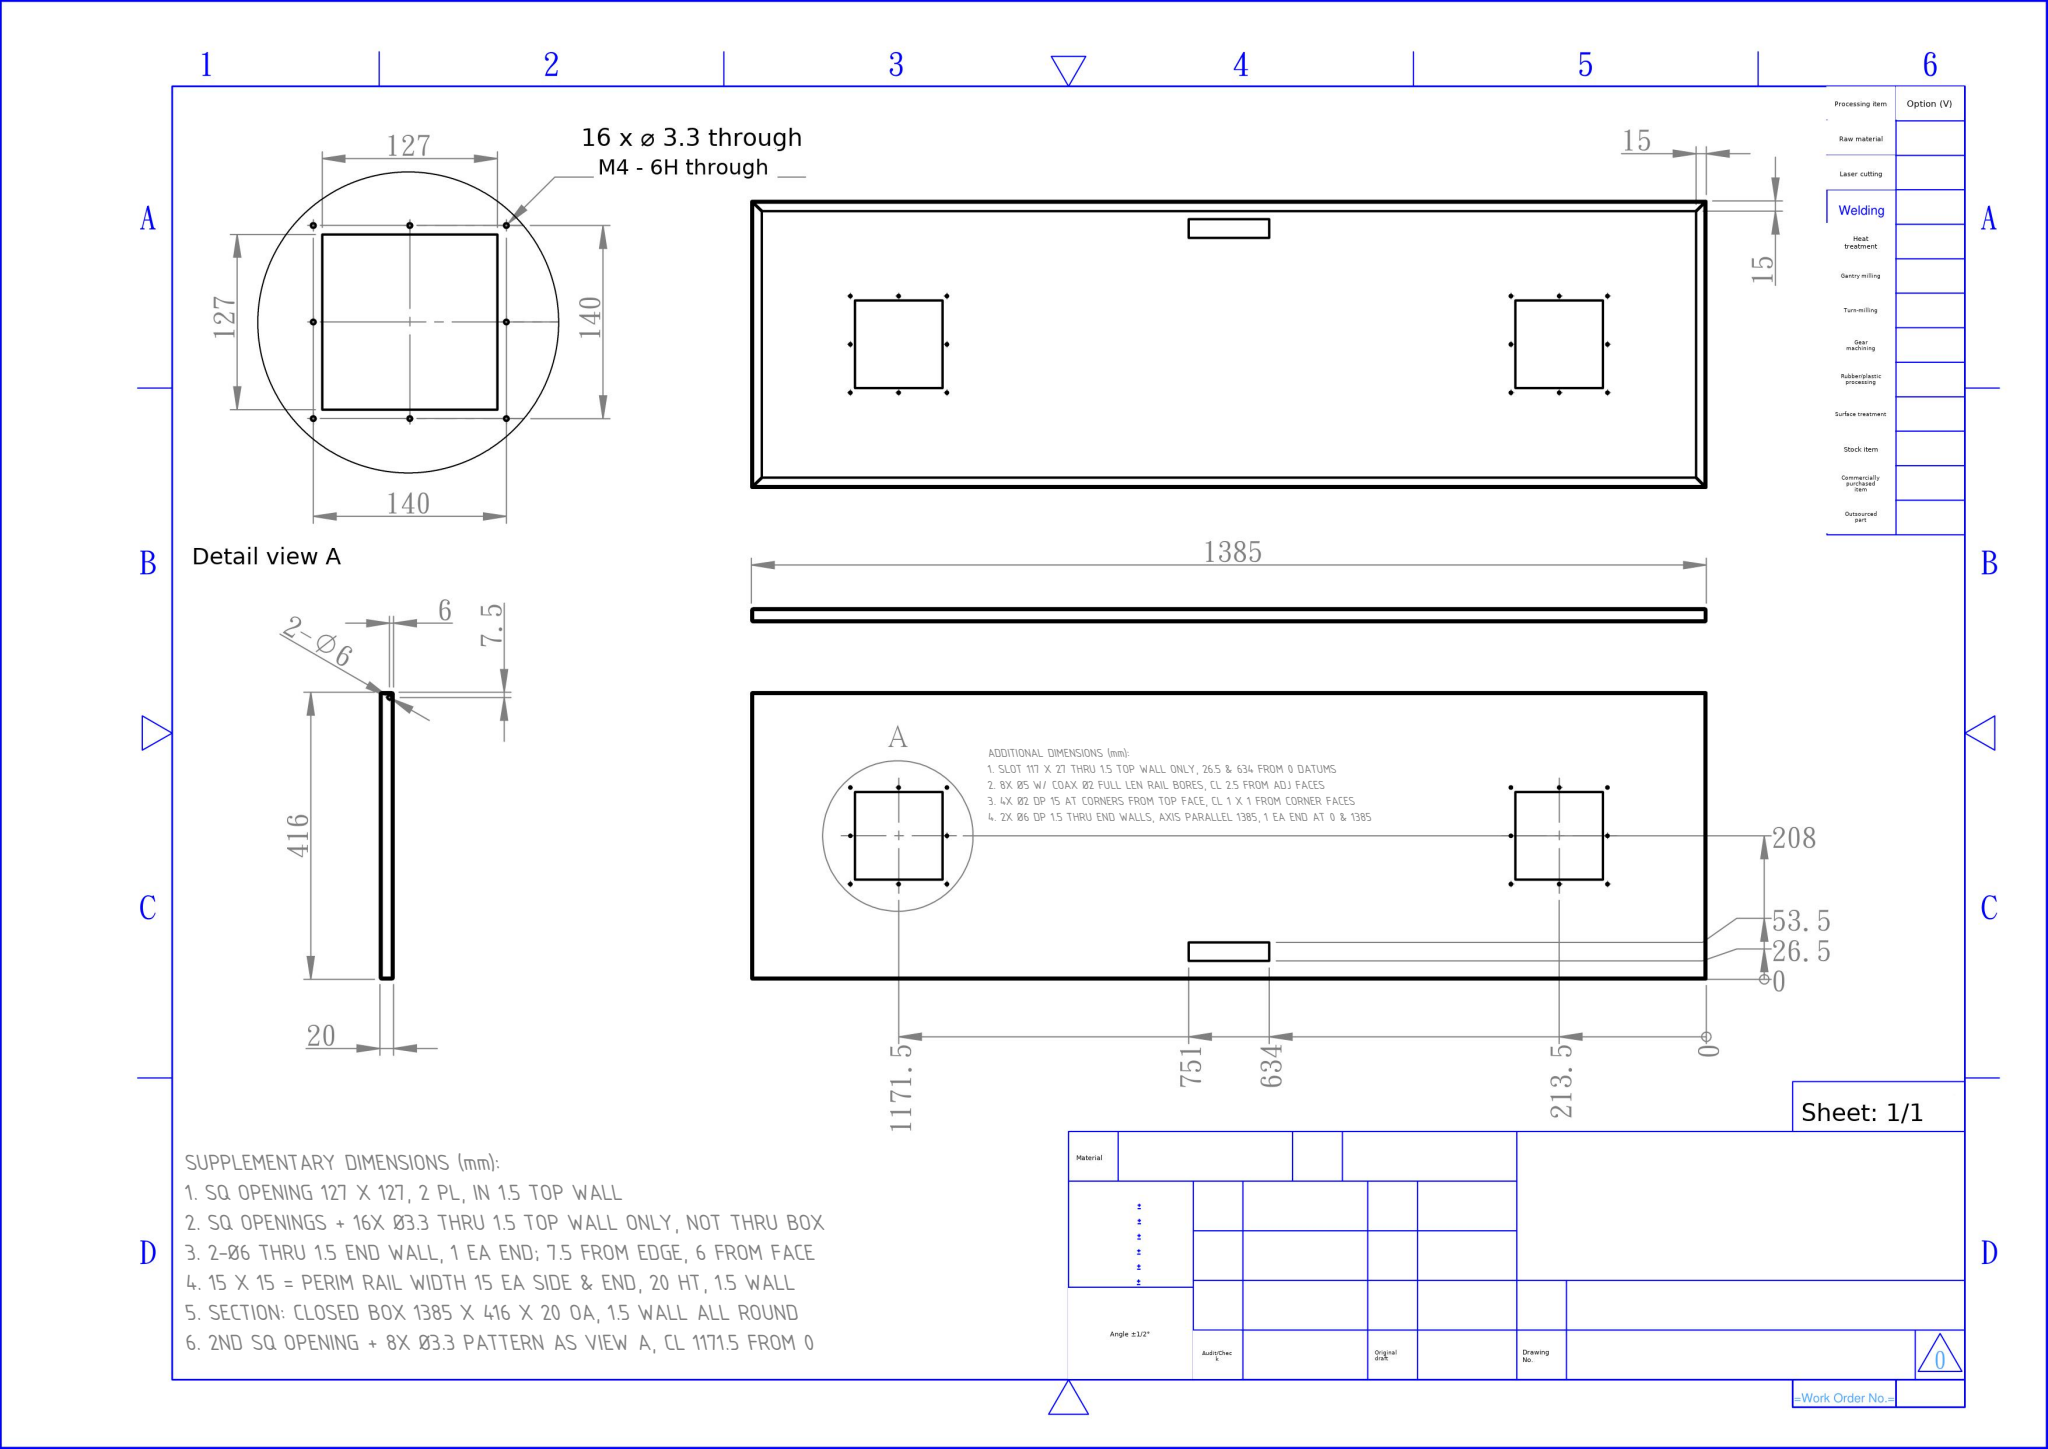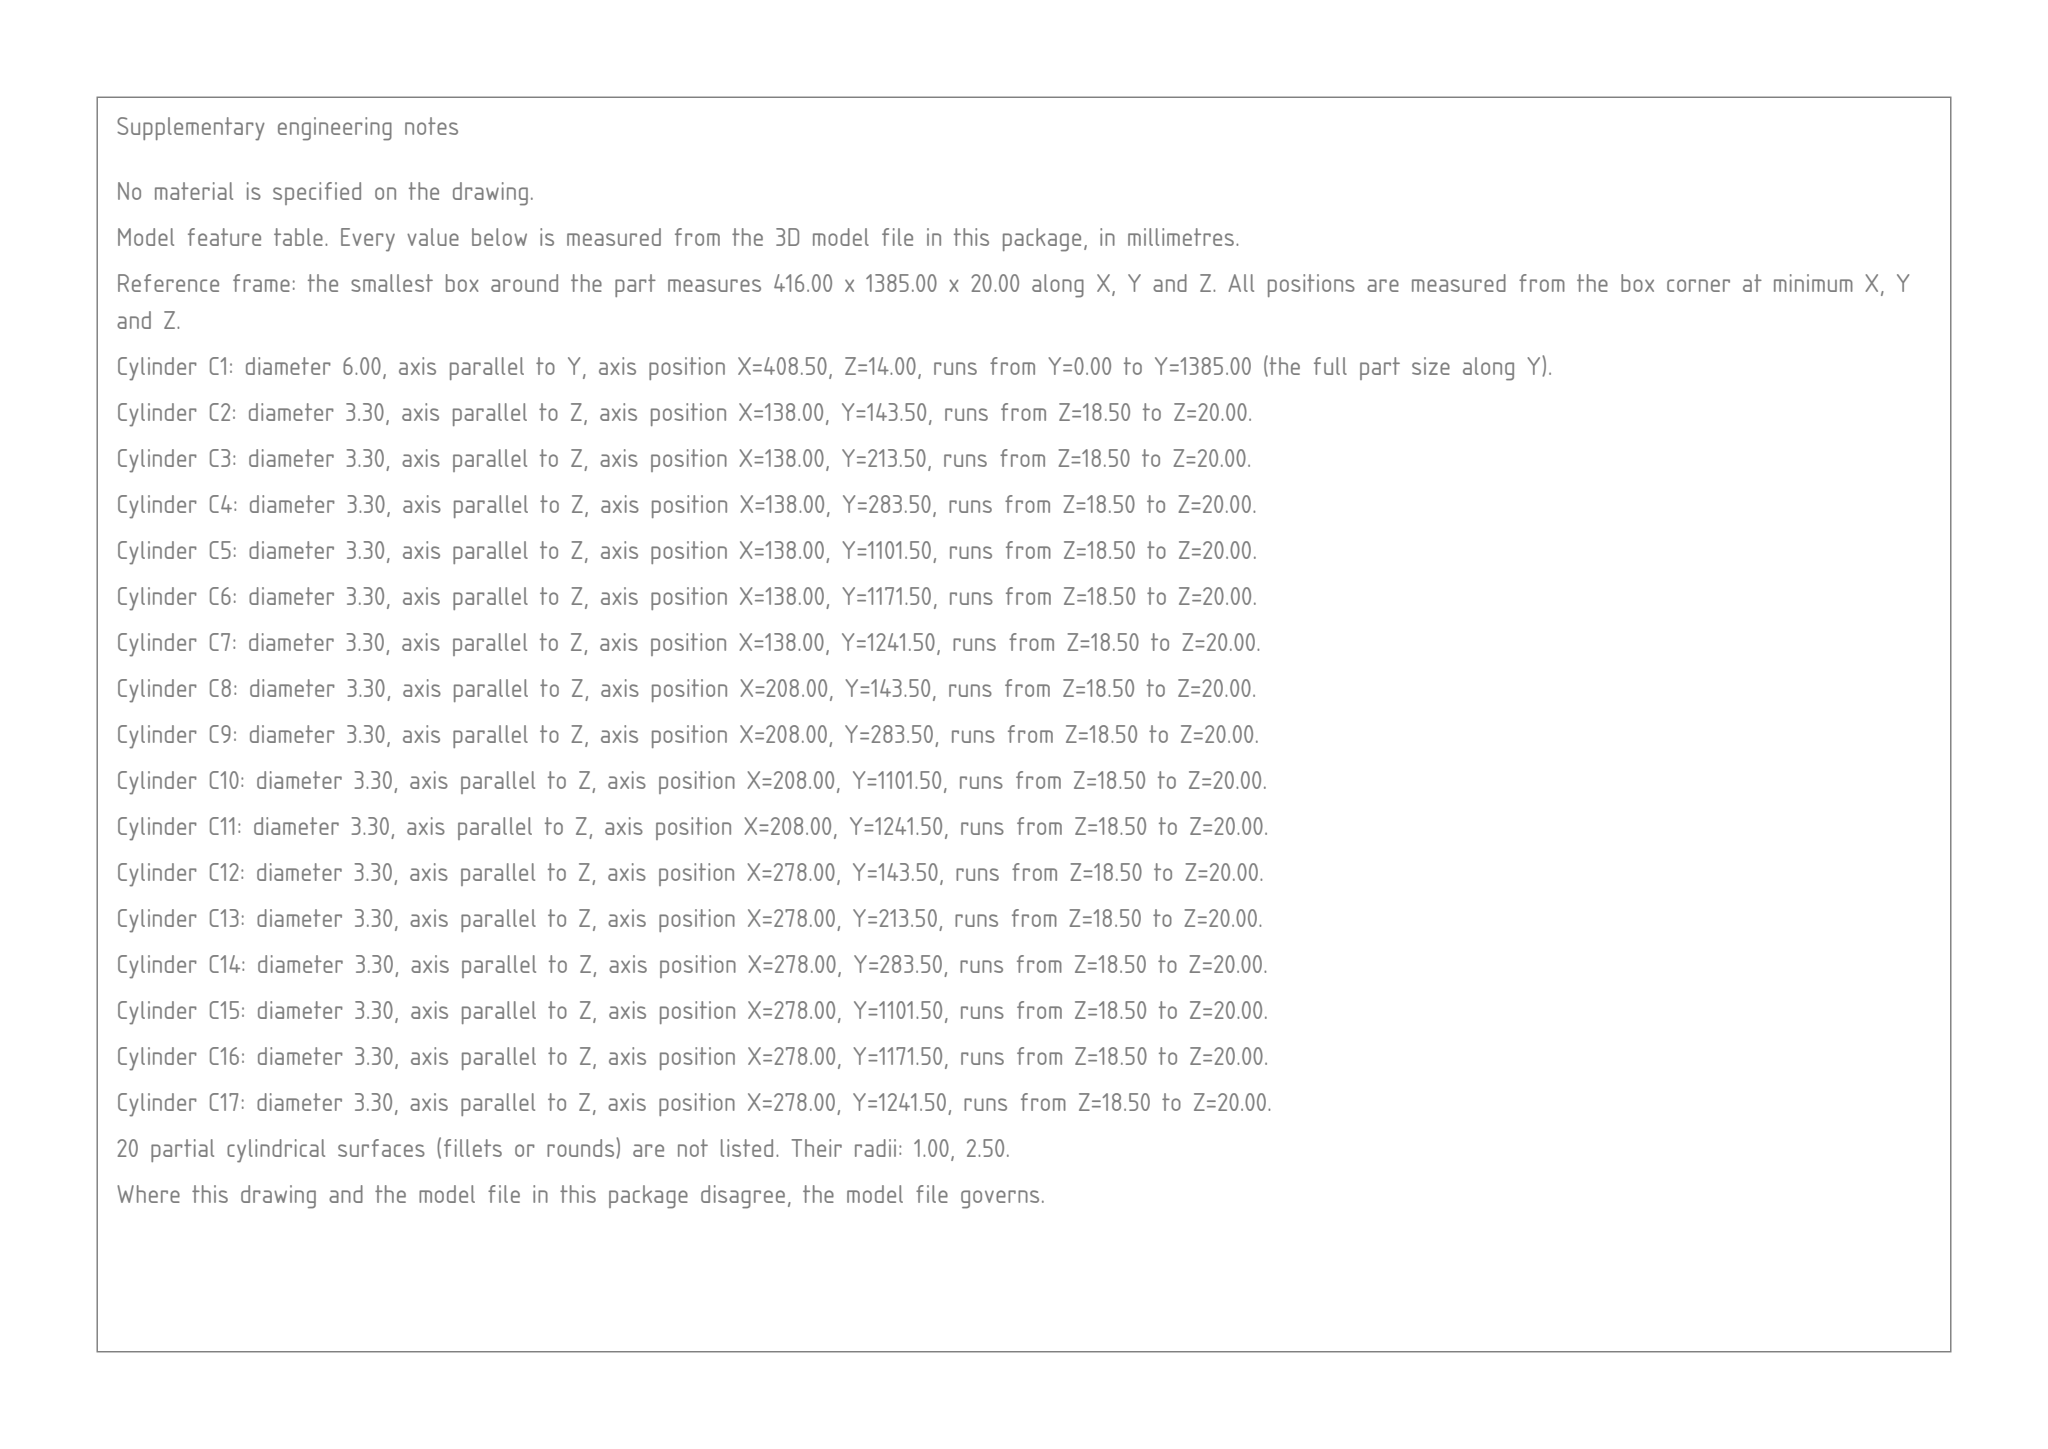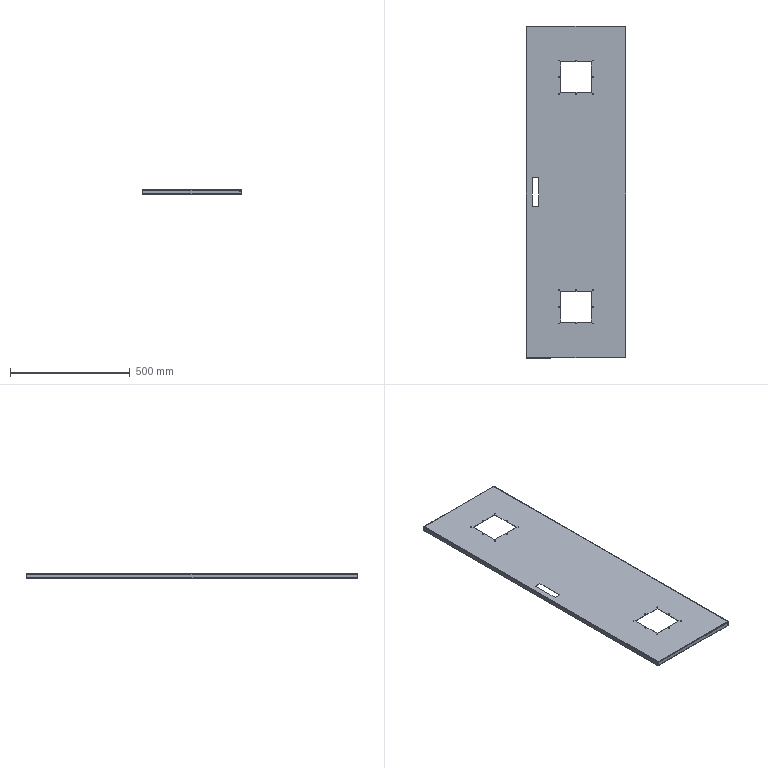Part | SolidWorks | mm | 1 solid | 162 faces | box 416 x 1385 x 20 mm | volume 974092 mm3 | plane 66 | cylinder 56 | spline 40 | commonest cylinder face diameters 3.3 x32 2 x12 5 x8 6 x4